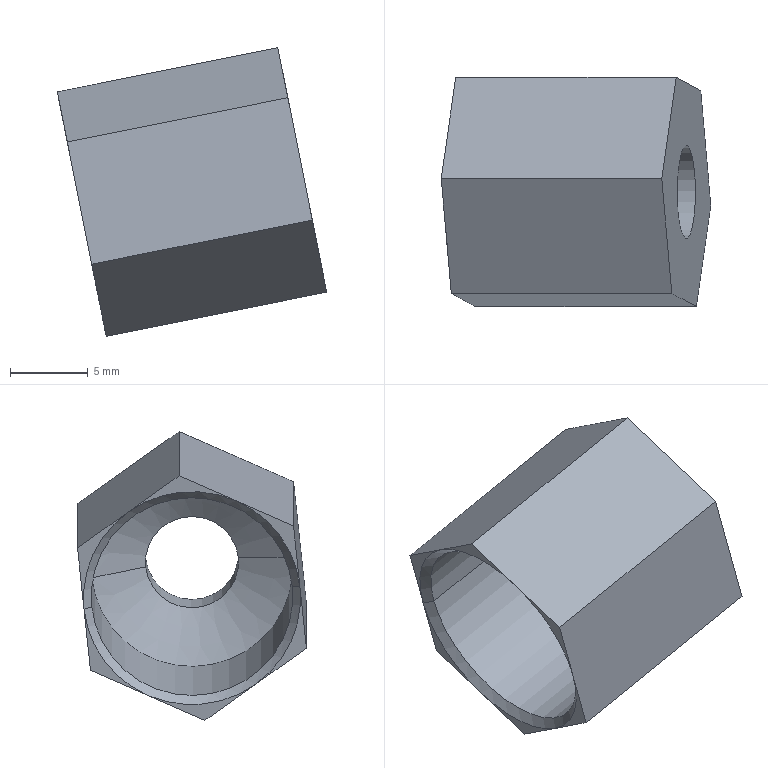Component | SolidWorks | 2-1 | 1 solid | 21 faces | box 17.38 x 14.76 x 18.62 mm | volume 920 mm3 | plane 13 | cone 4 | cylinder 4 | commonest cylinder face diameters 13 x2 6 x2
STEP:
#1=COLOUR_RGB('',0.7922,0.8196,0.9333);
#2=FILL_AREA_STYLE_COLOUR('',#1);
#3=FILL_AREA_STYLE('',(#2));
#4=SURFACE_STYLE_FILL_AREA(#3);
#5=SURFACE_SIDE_STYLE('',(#4));
#6=SURFACE_STYLE_USAGE(.BOTH.,#5);
#7=PRESENTATION_STYLE_ASSIGNMENT((#6));
#8=CARTESIAN_POINT('',(2.804,-12.312,0.535));
#9=VERTEX_POINT('',#8);
#10=CARTESIAN_POINT('',(2.793,-12.821,0.5869));
#11=VERTEX_POINT('',#10);
#12=CARTESIAN_POINT('',(2.799,-12.567,0.5609));
#13=DIRECTION('',(-0.9805,-0.,-0.1965));
#14=DIRECTION('',(-0.0203,-0.9947,0.1013));
#15=AXIS2_PLACEMENT_3D('',#12,#13,#14);
#16=CIRCLE('',#15,0.2559);
#17=EDGE_CURVE('',#9,#11,#16,.T.);
#18=ORIENTED_EDGE('',*,*,#17,.F.);
#19=CARTESIAN_POINT('',(2.785,-12.293,0.5292));
#20=VERTEX_POINT('',#19);
#21=CARTESIAN_POINT('',(2.804,-12.312,0.535));
#22=DIRECTION('',(-0.679,0.7033,-0.2106));
#23=VECTOR('',#22,39.37);
#24=LINE('',#21,#23);
#25=EDGE_CURVE('',#9,#20,#24,.T.);
#26=ORIENTED_EDGE('',*,*,#25,.T.);
#27=CARTESIAN_POINT('',(2.829,-12.455,0.3103));
#28=VERTEX_POINT('',#27);
#29=CARTESIAN_POINT('',(2.779,-12.567,0.5571));
#30=DIRECTION('',(0.9805,0.,0.1965));
#31=DIRECTION('',(-0.0203,-0.9947,0.1013));
#32=AXIS2_PLACEMENT_3D('',#29,#30,#31);
#33=CIRCLE('',#32,0.2756);
#34=EDGE_CURVE('',#28,#20,#33,.T.);
#35=ORIENTED_EDGE('',*,*,#34,.F.);
#36=CARTESIAN_POINT('',(2.823,-12.729,0.3383));
#37=VERTEX_POINT('',#36);
#38=CARTESIAN_POINT('',(2.779,-12.567,0.5571));
#39=DIRECTION('',(0.9805,0.,0.1965));
#40=DIRECTION('',(-0.0203,-0.9947,0.1013));
#41=AXIS2_PLACEMENT_3D('',#38,#39,#40);
#42=CIRCLE('',#41,0.2756);
#43=EDGE_CURVE('',#37,#28,#42,.T.);
#44=ORIENTED_EDGE('',*,*,#43,.F.);
#45=CARTESIAN_POINT('',(2.774,-12.841,0.585));
#46=VERTEX_POINT('',#45);
#47=CARTESIAN_POINT('',(2.779,-12.567,0.5571));
#48=DIRECTION('',(0.9805,0.,0.1965));
#49=DIRECTION('',(-0.0203,-0.9947,0.1013));
#50=AXIS2_PLACEMENT_3D('',#47,#48,#49);
#51=CIRCLE('',#50,0.2756);
#52=EDGE_CURVE('',#46,#37,#51,.T.);
#53=ORIENTED_EDGE('',*,*,#52,.F.);
#54=CARTESIAN_POINT('',(2.793,-12.821,0.5869));
#55=DIRECTION('',(-0.7077,-0.7033,-0.06734));
#56=VECTOR('',#55,39.37);
#57=LINE('',#54,#56);
#58=EDGE_CURVE('',#11,#46,#57,.T.);
#59=ORIENTED_EDGE('',*,*,#58,.F.);
#60=EDGE_LOOP('',(#18,#26,#35,#44,#53,#59));
#61=FACE_OUTER_BOUND('',#60,.T.);
#62=CARTESIAN_POINT('',(2.799,-12.567,0.5609));
#63=DIRECTION('',(-0.9805,-0.,-0.1965));
#64=DIRECTION('',(-0.0203,-0.9947,0.1013));
#65=AXIS2_PLACEMENT_3D('',#62,#63,#64);
#66=CONICAL_SURFACE('',#65,0.2559,0.7854);
#67=ADVANCED_FACE('',(#61),#66,.F.);
#68=CARTESIAN_POINT('',(3.171,-12.312,0.6085));
#69=VERTEX_POINT('',#68);
#70=CARTESIAN_POINT('',(3.16,-12.821,0.6604));
#71=VERTEX_POINT('',#70);
#72=CARTESIAN_POINT('',(3.165,-12.567,0.6344));
#73=DIRECTION('',(-0.9805,-0.,-0.1965));
#74=DIRECTION('',(-0.0203,-0.9947,0.1013));
#75=AXIS2_PLACEMENT_3D('',#72,#73,#74);
#76=CIRCLE('',#75,0.2559);
#77=EDGE_CURVE('',#69,#71,#76,.T.);
#78=ORIENTED_EDGE('',*,*,#77,.F.);
#79=CARTESIAN_POINT('',(2.785,-12.312,0.5311));
#80=DIRECTION('',(-0.9805,-0.,-0.1965));
#81=VECTOR('',#80,39.37);
#82=LINE('',#79,#81);
#83=EDGE_CURVE('',#69,#9,#82,.T.);
#84=ORIENTED_EDGE('',*,*,#83,.T.);
#85=ORIENTED_EDGE('',*,*,#17,.T.);
#86=CARTESIAN_POINT('',(2.774,-12.821,0.583));
#87=DIRECTION('',(-0.9805,-0.,-0.1965));
#88=VECTOR('',#87,39.37);
#89=LINE('',#86,#88);
#90=EDGE_CURVE('',#71,#11,#89,.T.);
#91=ORIENTED_EDGE('',*,*,#90,.F.);
#92=EDGE_LOOP('',(#78,#84,#85,#91));
#93=FACE_OUTER_BOUND('',#92,.T.);
#94=CARTESIAN_POINT('',(2.779,-12.567,0.5571));
#95=DIRECTION('',(-0.9805,-0.,-0.1965));
#96=DIRECTION('',(-0.0203,-0.9947,0.1013));
#97=AXIS2_PLACEMENT_3D('',#94,#95,#96);
#98=CYLINDRICAL_SURFACE('',#97,0.2559);
#99=ADVANCED_FACE('',(#93),#98,.F.);
#100=CARTESIAN_POINT('',(3.237,-12.449,0.6363));
#101=VERTEX_POINT('',#100);
#102=CARTESIAN_POINT('',(3.232,-12.684,0.6602));
#103=VERTEX_POINT('',#102);
#104=CARTESIAN_POINT('',(3.234,-12.567,0.6482));
#105=DIRECTION('',(-0.9805,-0.,-0.1965));
#106=DIRECTION('',(-0.0203,-0.9947,0.1013));
#107=AXIS2_PLACEMENT_3D('',#104,#105,#106);
#108=CIRCLE('',#107,0.1181);
#109=EDGE_CURVE('',#101,#103,#108,.T.);
#110=ORIENTED_EDGE('',*,*,#109,.F.);
#111=CARTESIAN_POINT('',(3.171,-12.312,0.6085));
#112=DIRECTION('',(-0.427,0.8862,-0.1795));
#113=VECTOR('',#112,39.37);
#114=LINE('',#111,#113);
#115=EDGE_CURVE('',#101,#69,#114,.T.);
#116=ORIENTED_EDGE('',*,*,#115,.T.);
#117=ORIENTED_EDGE('',*,*,#77,.T.);
#118=CARTESIAN_POINT('',(3.16,-12.821,0.6604));
#119=DIRECTION('',(-0.4632,-0.8862,0.001028));
#120=VECTOR('',#119,39.37);
#121=LINE('',#118,#120);
#122=EDGE_CURVE('',#103,#71,#121,.T.);
#123=ORIENTED_EDGE('',*,*,#122,.F.);
#124=EDGE_LOOP('',(#110,#116,#117,#123));
#125=FACE_OUTER_BOUND('',#124,.T.);
#126=CARTESIAN_POINT('',(3.165,-12.567,0.6344));
#127=DIRECTION('',(-0.9805,-0.,-0.1965));
#128=DIRECTION('',(-0.0203,-0.9947,0.1013));
#129=AXIS2_PLACEMENT_3D('',#126,#127,#128);
#130=CONICAL_SURFACE('',#129,0.2559,1.1);
#131=ADVANCED_FACE('',(#125),#130,.F.);
#132=CARTESIAN_POINT('',(3.342,-12.449,0.6573));
#133=VERTEX_POINT('',#132);
#134=CARTESIAN_POINT('',(3.337,-12.684,0.6812));
#135=VERTEX_POINT('',#134);
#136=CARTESIAN_POINT('',(3.339,-12.567,0.6693));
#137=DIRECTION('',(-0.9805,-0.,-0.1965));
#138=DIRECTION('',(-0.0203,-0.9947,0.1013));
#139=AXIS2_PLACEMENT_3D('',#136,#137,#138);
#140=CIRCLE('',#139,0.1181);
#141=EDGE_CURVE('',#133,#135,#140,.T.);
#142=ORIENTED_EDGE('',*,*,#141,.F.);
#143=CARTESIAN_POINT('',(2.782,-12.449,0.5451));
#144=DIRECTION('',(-0.9805,-0.,-0.1965));
#145=VECTOR('',#144,39.37);
#146=LINE('',#143,#145);
#147=EDGE_CURVE('',#133,#101,#146,.T.);
#148=ORIENTED_EDGE('',*,*,#147,.T.);
#149=ORIENTED_EDGE('',*,*,#109,.T.);
#150=CARTESIAN_POINT('',(2.777,-12.684,0.569));
#151=DIRECTION('',(-0.9805,-0.,-0.1965));
#152=VECTOR('',#151,39.37);
#153=LINE('',#150,#152);
#154=EDGE_CURVE('',#135,#103,#153,.T.);
#155=ORIENTED_EDGE('',*,*,#154,.F.);
#156=EDGE_LOOP('',(#142,#148,#149,#155));
#157=FACE_OUTER_BOUND('',#156,.T.);
#158=CARTESIAN_POINT('',(2.779,-12.567,0.5571));
#159=DIRECTION('',(-0.9805,-0.,-0.1965));
#160=DIRECTION('',(-0.0203,-0.9947,0.1013));
#161=AXIS2_PLACEMENT_3D('',#158,#159,#160);
#162=CYLINDRICAL_SURFACE('',#161,0.1181);
#163=ADVANCED_FACE('',(#157),#162,.F.);
#164=CARTESIAN_POINT('',(2.805,-12.857,0.4298));
#165=VERTEX_POINT('',#164);
#166=CARTESIAN_POINT('',(2.805,-12.857,0.4298));
#167=DIRECTION('',(-0.1955,0.1033,0.9753));
#168=VECTOR('',#167,39.37);
#169=LINE('',#166,#168);
#170=EDGE_CURVE('',#165,#46,#169,.T.);
#171=ORIENTED_EDGE('',*,*,#170,.T.);
#172=ORIENTED_EDGE('',*,*,#52,.T.);
#173=CARTESIAN_POINT('',(2.842,-12.6,0.2467));
#174=DIRECTION('',(-0.1153,-0.8097,0.5753));
#175=VECTOR('',#174,39.37);
#176=LINE('',#173,#175);
#177=EDGE_CURVE('',#37,#165,#176,.T.);
#178=ORIENTED_EDGE('',*,*,#177,.T.);
#179=EDGE_LOOP('',(#171,#172,#178));
#180=FACE_OUTER_BOUND('',#179,.T.);
#181=CARTESIAN_POINT('',(2.779,-12.567,0.5571));
#182=DIRECTION('',(-0.9805,-0.,-0.1965));
#183=DIRECTION('',(-0.0203,-0.9947,0.1013));
#184=AXIS2_PLACEMENT_3D('',#181,#182,#183);
#185=PLANE('',#184);
#186=ADVANCED_FACE('',(#180),#185,.T.);
#187=CARTESIAN_POINT('',(2.842,-12.6,0.2467));
#188=VERTEX_POINT('',#187);
#189=CARTESIAN_POINT('',(2.842,-12.6,0.2467));
#190=DIRECTION('',(-0.1153,-0.8097,0.5753));
#191=VECTOR('',#190,39.37);
#192=LINE('',#189,#191);
#193=EDGE_CURVE('',#188,#37,#192,.T.);
#194=ORIENTED_EDGE('',*,*,#193,.T.);
#195=ORIENTED_EDGE('',*,*,#43,.T.);
#196=CARTESIAN_POINT('',(2.816,-12.309,0.374));
#197=DIRECTION('',(0.08015,-0.913,-0.3999));
#198=VECTOR('',#197,39.37);
#199=LINE('',#196,#198);
#200=EDGE_CURVE('',#28,#188,#199,.T.);
#201=ORIENTED_EDGE('',*,*,#200,.T.);
#202=EDGE_LOOP('',(#194,#195,#201));
#203=FACE_OUTER_BOUND('',#202,.T.);
#204=CARTESIAN_POINT('',(2.779,-12.567,0.5571));
#205=DIRECTION('',(-0.9805,-0.,-0.1965));
#206=DIRECTION('',(-0.0203,-0.9947,0.1013));
#207=AXIS2_PLACEMENT_3D('',#204,#205,#206);
#208=PLANE('',#207);
#209=ADVANCED_FACE('',(#203),#208,.T.);
#210=CARTESIAN_POINT('',(2.816,-12.309,0.374));
#211=VERTEX_POINT('',#210);
#212=CARTESIAN_POINT('',(2.816,-12.309,0.374));
#213=DIRECTION('',(0.08015,-0.913,-0.3999));
#214=VECTOR('',#213,39.37);
#215=LINE('',#212,#214);
#216=EDGE_CURVE('',#211,#28,#215,.T.);
#217=ORIENTED_EDGE('',*,*,#216,.T.);
#218=ORIENTED_EDGE('',*,*,#34,.T.);
#219=CARTESIAN_POINT('',(2.754,-12.276,0.6843));
#220=DIRECTION('',(0.1955,-0.1033,-0.9753));
#221=VECTOR('',#220,39.37);
#222=LINE('',#219,#221);
#223=EDGE_CURVE('',#20,#211,#222,.T.);
#224=ORIENTED_EDGE('',*,*,#223,.T.);
#225=EDGE_LOOP('',(#217,#218,#224));
#226=FACE_OUTER_BOUND('',#225,.T.);
#227=CARTESIAN_POINT('',(2.779,-12.567,0.5571));
#228=DIRECTION('',(-0.9805,-0.,-0.1965));
#229=DIRECTION('',(-0.0203,-0.9947,0.1013));
#230=AXIS2_PLACEMENT_3D('',#227,#228,#229);
#231=PLANE('',#230);
#232=ADVANCED_FACE('',(#226),#231,.T.);
#233=CARTESIAN_POINT('',(2.754,-12.276,0.6843));
#234=VERTEX_POINT('',#233);
#235=CARTESIAN_POINT('',(2.754,-12.276,0.6843));
#236=DIRECTION('',(0.1955,-0.1033,-0.9753));
#237=VECTOR('',#236,39.37);
#238=LINE('',#235,#237);
#239=EDGE_CURVE('',#234,#20,#238,.T.);
#240=ORIENTED_EDGE('',*,*,#239,.T.);
#241=CARTESIAN_POINT('',(2.736,-12.405,0.7759));
#242=VERTEX_POINT('',#241);
#243=CARTESIAN_POINT('',(2.779,-12.567,0.5571));
#244=DIRECTION('',(0.9805,0.,0.1965));
#245=DIRECTION('',(-0.0203,-0.9947,0.1013));
#246=AXIS2_PLACEMENT_3D('',#243,#244,#245);
#247=CIRCLE('',#246,0.2756);
#248=EDGE_CURVE('',#20,#242,#247,.T.);
#249=ORIENTED_EDGE('',*,*,#248,.T.);
#250=CARTESIAN_POINT('',(2.717,-12.534,0.8674));
#251=DIRECTION('',(0.1153,0.8097,-0.5753));
#252=VECTOR('',#251,39.37);
#253=LINE('',#250,#252);
#254=EDGE_CURVE('',#242,#234,#253,.T.);
#255=ORIENTED_EDGE('',*,*,#254,.T.);
#256=EDGE_LOOP('',(#240,#249,#255));
#257=FACE_OUTER_BOUND('',#256,.T.);
#258=CARTESIAN_POINT('',(2.779,-12.567,0.5571));
#259=DIRECTION('',(-0.9805,-0.,-0.1965));
#260=DIRECTION('',(-0.0203,-0.9947,0.1013));
#261=AXIS2_PLACEMENT_3D('',#258,#259,#260);
#262=PLANE('',#261);
#263=ADVANCED_FACE('',(#257),#262,.T.);
#264=CARTESIAN_POINT('',(2.717,-12.534,0.8674));
#265=VERTEX_POINT('',#264);
#266=CARTESIAN_POINT('',(2.717,-12.534,0.8674));
#267=DIRECTION('',(0.1153,0.8097,-0.5753));
#268=VECTOR('',#267,39.37);
#269=LINE('',#266,#268);
#270=EDGE_CURVE('',#265,#242,#269,.T.);
#271=ORIENTED_EDGE('',*,*,#270,.T.);
#272=CARTESIAN_POINT('',(2.73,-12.679,0.8038));
#273=VERTEX_POINT('',#272);
#274=CARTESIAN_POINT('',(2.779,-12.567,0.5571));
#275=DIRECTION('',(0.9805,0.,0.1965));
#276=DIRECTION('',(-0.0203,-0.9947,0.1013));
#277=AXIS2_PLACEMENT_3D('',#274,#275,#276);
#278=CIRCLE('',#277,0.2756);
#279=EDGE_CURVE('',#242,#273,#278,.T.);
#280=ORIENTED_EDGE('',*,*,#279,.T.);
#281=CARTESIAN_POINT('',(2.743,-12.825,0.7402));
#282=DIRECTION('',(-0.08015,0.913,0.3999));
#283=VECTOR('',#282,39.37);
#284=LINE('',#281,#283);
#285=EDGE_CURVE('',#273,#265,#284,.T.);
#286=ORIENTED_EDGE('',*,*,#285,.T.);
#287=EDGE_LOOP('',(#271,#280,#286));
#288=FACE_OUTER_BOUND('',#287,.T.);
#289=CARTESIAN_POINT('',(2.779,-12.567,0.5571));
#290=DIRECTION('',(-0.9805,-0.,-0.1965));
#291=DIRECTION('',(-0.0203,-0.9947,0.1013));
#292=AXIS2_PLACEMENT_3D('',#289,#290,#291);
#293=PLANE('',#292);
#294=ADVANCED_FACE('',(#288),#293,.T.);
#295=CARTESIAN_POINT('',(3.277,-12.534,0.9796));
#296=VERTEX_POINT('',#295);
#297=CARTESIAN_POINT('',(3.314,-12.276,0.7965));
#298=VERTEX_POINT('',#297);
#299=CARTESIAN_POINT('',(3.277,-12.534,0.9796));
#300=DIRECTION('',(0.1153,0.8097,-0.5753));
#301=VECTOR('',#300,39.37);
#302=LINE('',#299,#301);
#303=EDGE_CURVE('',#296,#298,#302,.T.);
#304=ORIENTED_EDGE('',*,*,#303,.T.);
#305=CARTESIAN_POINT('',(2.754,-12.276,0.6843));
#306=DIRECTION('',(0.9805,0.,0.1965));
#307=VECTOR('',#306,39.37);
#308=LINE('',#305,#307);
#309=EDGE_CURVE('',#234,#298,#308,.T.);
#310=ORIENTED_EDGE('',*,*,#309,.F.);
#311=ORIENTED_EDGE('',*,*,#254,.F.);
#312=ORIENTED_EDGE('',*,*,#270,.F.);
#313=CARTESIAN_POINT('',(2.717,-12.534,0.8674));
#314=DIRECTION('',(0.9805,0.,0.1965));
#315=VECTOR('',#314,39.37);
#316=LINE('',#313,#315);
#317=EDGE_CURVE('',#265,#296,#316,.T.);
#318=ORIENTED_EDGE('',*,*,#317,.T.);
#319=EDGE_LOOP('',(#304,#310,#311,#312,#318));
#320=FACE_OUTER_BOUND('',#319,.T.);
#321=CARTESIAN_POINT('',(2.717,-12.534,0.8674));
#322=DIRECTION('',(0.1591,-0.5868,-0.794));
#323=DIRECTION('',(-0.1153,-0.8097,0.5753));
#324=AXIS2_PLACEMENT_3D('',#321,#322,#323);
#325=PLANE('',#324);
#326=ADVANCED_FACE('',(#320),#325,.F.);
#327=CARTESIAN_POINT('',(3.376,-12.309,0.4862));
#328=VERTEX_POINT('',#327);
#329=CARTESIAN_POINT('',(3.314,-12.276,0.7965));
#330=DIRECTION('',(0.1955,-0.1033,-0.9753));
#331=VECTOR('',#330,39.37);
#332=LINE('',#329,#331);
#333=EDGE_CURVE('',#298,#328,#332,.T.);
#334=ORIENTED_EDGE('',*,*,#333,.T.);
#335=CARTESIAN_POINT('',(2.816,-12.309,0.374));
#336=DIRECTION('',(0.9805,0.,0.1965));
#337=VECTOR('',#336,39.37);
#338=LINE('',#335,#337);
#339=EDGE_CURVE('',#211,#328,#338,.T.);
#340=ORIENTED_EDGE('',*,*,#339,.F.);
#341=ORIENTED_EDGE('',*,*,#223,.F.);
#342=ORIENTED_EDGE('',*,*,#239,.F.);
#343=ORIENTED_EDGE('',*,*,#309,.T.);
#344=EDGE_LOOP('',(#334,#340,#341,#342,#343));
#345=FACE_OUTER_BOUND('',#344,.T.);
#346=CARTESIAN_POINT('',(2.754,-12.276,0.6843));
#347=DIRECTION('',(-0.0203,-0.9947,0.1013));
#348=DIRECTION('',(-0.1955,0.1033,0.9753));
#349=AXIS2_PLACEMENT_3D('',#346,#347,#348);
#350=PLANE('',#349);
#351=ADVANCED_FACE('',(#345),#350,.F.);
#352=CARTESIAN_POINT('',(3.401,-12.6,0.3589));
#353=VERTEX_POINT('',#352);
#354=CARTESIAN_POINT('',(3.376,-12.309,0.4862));
#355=DIRECTION('',(0.08015,-0.913,-0.3999));
#356=VECTOR('',#355,39.37);
#357=LINE('',#354,#356);
#358=EDGE_CURVE('',#328,#353,#357,.T.);
#359=ORIENTED_EDGE('',*,*,#358,.T.);
#360=CARTESIAN_POINT('',(2.842,-12.6,0.2467));
#361=DIRECTION('',(0.9805,0.,0.1965));
#362=VECTOR('',#361,39.37);
#363=LINE('',#360,#362);
#364=EDGE_CURVE('',#188,#353,#363,.T.);
#365=ORIENTED_EDGE('',*,*,#364,.F.);
#366=ORIENTED_EDGE('',*,*,#200,.F.);
#367=ORIENTED_EDGE('',*,*,#216,.F.);
#368=ORIENTED_EDGE('',*,*,#339,.T.);
#369=EDGE_LOOP('',(#359,#365,#366,#367,#368));
#370=FACE_OUTER_BOUND('',#369,.T.);
#371=CARTESIAN_POINT('',(2.816,-12.309,0.374));
#372=DIRECTION('',(-0.1794,-0.4079,0.8952));
#373=DIRECTION('',(-0.08015,0.913,0.3999));
#374=AXIS2_PLACEMENT_3D('',#371,#372,#373);
#375=PLANE('',#374);
#376=ADVANCED_FACE('',(#370),#375,.F.);
#377=CARTESIAN_POINT('',(3.365,-12.857,0.542));
#378=VERTEX_POINT('',#377);
#379=CARTESIAN_POINT('',(3.401,-12.6,0.3589));
#380=DIRECTION('',(-0.1153,-0.8097,0.5753));
#381=VECTOR('',#380,39.37);
#382=LINE('',#379,#381);
#383=EDGE_CURVE('',#353,#378,#382,.T.);
#384=ORIENTED_EDGE('',*,*,#383,.T.);
#385=CARTESIAN_POINT('',(2.805,-12.857,0.4298));
#386=DIRECTION('',(0.9805,0.,0.1965));
#387=VECTOR('',#386,39.37);
#388=LINE('',#385,#387);
#389=EDGE_CURVE('',#165,#378,#388,.T.);
#390=ORIENTED_EDGE('',*,*,#389,.F.);
#391=ORIENTED_EDGE('',*,*,#177,.F.);
#392=ORIENTED_EDGE('',*,*,#193,.F.);
#393=ORIENTED_EDGE('',*,*,#364,.T.);
#394=EDGE_LOOP('',(#384,#390,#391,#392,#393));
#395=FACE_OUTER_BOUND('',#394,.T.);
#396=CARTESIAN_POINT('',(2.842,-12.6,0.2467));
#397=DIRECTION('',(-0.1591,0.5868,0.794));
#398=DIRECTION('',(0.1153,0.8097,-0.5753));
#399=AXIS2_PLACEMENT_3D('',#396,#397,#398);
#400=PLANE('',#399);
#401=ADVANCED_FACE('',(#395),#400,.F.);
#402=CARTESIAN_POINT('',(3.302,-12.825,0.8523));
#403=VERTEX_POINT('',#402);
#404=CARTESIAN_POINT('',(3.365,-12.857,0.542));
#405=DIRECTION('',(-0.1955,0.1033,0.9753));
#406=VECTOR('',#405,39.37);
#407=LINE('',#404,#406);
#408=EDGE_CURVE('',#378,#403,#407,.T.);
#409=ORIENTED_EDGE('',*,*,#408,.T.);
#410=CARTESIAN_POINT('',(2.743,-12.825,0.7402));
#411=VERTEX_POINT('',#410);
#412=CARTESIAN_POINT('',(2.743,-12.825,0.7402));
#413=DIRECTION('',(0.9805,0.,0.1965));
#414=VECTOR('',#413,39.37);
#415=LINE('',#412,#414);
#416=EDGE_CURVE('',#411,#403,#415,.T.);
#417=ORIENTED_EDGE('',*,*,#416,.F.);
#418=CARTESIAN_POINT('',(2.805,-12.857,0.4298));
#419=DIRECTION('',(-0.1955,0.1033,0.9753));
#420=VECTOR('',#419,39.37);
#421=LINE('',#418,#420);
#422=EDGE_CURVE('',#46,#411,#421,.T.);
#423=ORIENTED_EDGE('',*,*,#422,.F.);
#424=ORIENTED_EDGE('',*,*,#170,.F.);
#425=ORIENTED_EDGE('',*,*,#389,.T.);
#426=EDGE_LOOP('',(#409,#417,#423,#424,#425));
#427=FACE_OUTER_BOUND('',#426,.T.);
#428=CARTESIAN_POINT('',(2.805,-12.857,0.4298));
#429=DIRECTION('',(0.0203,0.9947,-0.1013));
#430=DIRECTION('',(0.1955,-0.1033,-0.9753));
#431=AXIS2_PLACEMENT_3D('',#428,#429,#430);
#432=PLANE('',#431);
#433=ADVANCED_FACE('',(#427),#432,.F.);
#434=CARTESIAN_POINT('',(3.302,-12.825,0.8523));
#435=DIRECTION('',(-0.08015,0.913,0.3999));
#436=VECTOR('',#435,39.37);
#437=LINE('',#434,#436);
#438=EDGE_CURVE('',#403,#296,#437,.T.);
#439=ORIENTED_EDGE('',*,*,#438,.T.);
#440=ORIENTED_EDGE('',*,*,#317,.F.);
#441=ORIENTED_EDGE('',*,*,#285,.F.);
#442=CARTESIAN_POINT('',(2.743,-12.825,0.7402));
#443=DIRECTION('',(-0.08015,0.913,0.3999));
#444=VECTOR('',#443,39.37);
#445=LINE('',#442,#444);
#446=EDGE_CURVE('',#411,#273,#445,.T.);
#447=ORIENTED_EDGE('',*,*,#446,.F.);
#448=ORIENTED_EDGE('',*,*,#416,.T.);
#449=EDGE_LOOP('',(#439,#440,#441,#447,#448));
#450=FACE_OUTER_BOUND('',#449,.T.);
#451=CARTESIAN_POINT('',(2.743,-12.825,0.7402));
#452=DIRECTION('',(0.1794,0.4079,-0.8952));
#453=DIRECTION('',(0.08015,-0.913,-0.3999));
#454=AXIS2_PLACEMENT_3D('',#451,#452,#453);
#455=PLANE('',#454);
#456=ADVANCED_FACE('',(#450),#455,.F.);
#457=ORIENTED_EDGE('',*,*,#446,.T.);
#458=CARTESIAN_POINT('',(2.779,-12.567,0.5571));
#459=DIRECTION('',(0.9805,0.,0.1965));
#460=DIRECTION('',(-0.0203,-0.9947,0.1013));
#461=AXIS2_PLACEMENT_3D('',#458,#459,#460);
#462=CIRCLE('',#461,0.2756);
#463=EDGE_CURVE('',#273,#46,#462,.T.);
#464=ORIENTED_EDGE('',*,*,#463,.T.);
#465=ORIENTED_EDGE('',*,*,#422,.T.);
#466=EDGE_LOOP('',(#457,#464,#465));
#467=FACE_OUTER_BOUND('',#466,.T.);
#468=CARTESIAN_POINT('',(2.779,-12.567,0.5571));
#469=DIRECTION('',(-0.9805,-0.,-0.1965));
#470=DIRECTION('',(-0.0203,-0.9947,0.1013));
#471=AXIS2_PLACEMENT_3D('',#468,#469,#470);
#472=PLANE('',#471);
#473=ADVANCED_FACE('',(#467),#472,.T.);
#474=CARTESIAN_POINT('',(3.339,-12.567,0.6693));
#475=DIRECTION('',(-0.9805,-0.,-0.1965));
#476=DIRECTION('',(-0.0203,-0.9947,0.1013));
#477=AXIS2_PLACEMENT_3D('',#474,#475,#476);
#478=CIRCLE('',#477,0.1181);
#479=EDGE_CURVE('',#135,#133,#478,.T.);
#480=ORIENTED_EDGE('',*,*,#479,.T.);
#481=ORIENTED_EDGE('',*,*,#141,.T.);
#482=EDGE_LOOP('',(#480,#481));
#483=FACE_BOUND('',#482,.T.);
#484=ORIENTED_EDGE('',*,*,#303,.F.);
#485=ORIENTED_EDGE('',*,*,#438,.F.);
#486=ORIENTED_EDGE('',*,*,#408,.F.);
#487=ORIENTED_EDGE('',*,*,#383,.F.);
#488=ORIENTED_EDGE('',*,*,#358,.F.);
#489=ORIENTED_EDGE('',*,*,#333,.F.);
#490=EDGE_LOOP('',(#484,#485,#486,#487,#488,#489));
#491=FACE_OUTER_BOUND('',#490,.T.);
#492=CARTESIAN_POINT('',(3.339,-12.567,0.6693));
#493=DIRECTION('',(-0.9805,-0.,-0.1965));
#494=DIRECTION('',(-0.0203,-0.9947,0.1013));
#495=AXIS2_PLACEMENT_3D('',#492,#493,#494);
#496=PLANE('',#495);
#497=ADVANCED_FACE('',(#483,#491),#496,.F.);
#498=ORIENTED_EDGE('',*,*,#147,.F.);
#499=ORIENTED_EDGE('',*,*,#479,.F.);
#500=ORIENTED_EDGE('',*,*,#154,.T.);
#501=CARTESIAN_POINT('',(3.234,-12.567,0.6482));
#502=DIRECTION('',(-0.9805,-0.,-0.1965));
#503=DIRECTION('',(-0.0203,-0.9947,0.1013));
#504=AXIS2_PLACEMENT_3D('',#501,#502,#503);
#505=CIRCLE('',#504,0.1181);
#506=EDGE_CURVE('',#103,#101,#505,.T.);
#507=ORIENTED_EDGE('',*,*,#506,.T.);
#508=EDGE_LOOP('',(#498,#499,#500,#507));
#509=FACE_OUTER_BOUND('',#508,.T.);
#510=CARTESIAN_POINT('',(2.779,-12.567,0.5571));
#511=DIRECTION('',(-0.9805,-0.,-0.1965));
#512=DIRECTION('',(-0.0203,-0.9947,0.1013));
#513=AXIS2_PLACEMENT_3D('',#510,#511,#512);
#514=CYLINDRICAL_SURFACE('',#513,0.1181);
#515=ADVANCED_FACE('',(#509),#514,.F.);
#516=ORIENTED_EDGE('',*,*,#115,.F.);
#517=ORIENTED_EDGE('',*,*,#506,.F.);
#518=ORIENTED_EDGE('',*,*,#122,.T.);
#519=CARTESIAN_POINT('',(3.165,-12.567,0.6344));
#520=DIRECTION('',(-0.9805,-0.,-0.1965));
#521=DIRECTION('',(-0.0203,-0.9947,0.1013));
#522=AXIS2_PLACEMENT_3D('',#519,#520,#521);
#523=CIRCLE('',#522,0.2559);
#524=EDGE_CURVE('',#71,#69,#523,.T.);
#525=ORIENTED_EDGE('',*,*,#524,.T.);
#526=EDGE_LOOP('',(#516,#517,#518,#525));
#527=FACE_OUTER_BOUND('',#526,.T.);
#528=CARTESIAN_POINT('',(3.165,-12.567,0.6344));
#529=DIRECTION('',(-0.9805,-0.,-0.1965));
#530=DIRECTION('',(-0.0203,-0.9947,0.1013));
#531=AXIS2_PLACEMENT_3D('',#528,#529,#530);
#532=CONICAL_SURFACE('',#531,0.2559,1.1);
#533=ADVANCED_FACE('',(#527),#532,.F.);
#534=ORIENTED_EDGE('',*,*,#83,.F.);
#535=ORIENTED_EDGE('',*,*,#524,.F.);
#536=ORIENTED_EDGE('',*,*,#90,.T.);
#537=CARTESIAN_POINT('',(2.799,-12.567,0.5609));
#538=DIRECTION('',(-0.9805,-0.,-0.1965));
#539=DIRECTION('',(-0.0203,-0.9947,0.1013));
#540=AXIS2_PLACEMENT_3D('',#537,#538,#539);
#541=CIRCLE('',#540,0.2559);
#542=EDGE_CURVE('',#11,#9,#541,.T.);
#543=ORIENTED_EDGE('',*,*,#542,.T.);
#544=EDGE_LOOP('',(#534,#535,#536,#543));
#545=FACE_OUTER_BOUND('',#544,.T.);
#546=CARTESIAN_POINT('',(2.779,-12.567,0.5571));
#547=DIRECTION('',(-0.9805,-0.,-0.1965));
#548=DIRECTION('',(-0.0203,-0.9947,0.1013));
#549=AXIS2_PLACEMENT_3D('',#546,#547,#548);
#550=CYLINDRICAL_SURFACE('',#549,0.2559);
#551=ADVANCED_FACE('',(#545),#550,.F.);
#552=ORIENTED_EDGE('',*,*,#25,.F.);
#553=ORIENTED_EDGE('',*,*,#542,.F.);
#554=ORIENTED_EDGE('',*,*,#58,.T.);
#555=ORIENTED_EDGE('',*,*,#463,.F.);
#556=ORIENTED_EDGE('',*,*,#279,.F.);
#557=ORIENTED_EDGE('',*,*,#248,.F.);
#558=EDGE_LOOP('',(#552,#553,#554,#555,#556,#557));
#559=FACE_OUTER_BOUND('',#558,.T.);
#560=CARTESIAN_POINT('',(2.799,-12.567,0.5609));
#561=DIRECTION('',(-0.9805,-0.,-0.1965));
#562=DIRECTION('',(-0.0203,-0.9947,0.1013));
#563=AXIS2_PLACEMENT_3D('',#560,#561,#562);
#564=CONICAL_SURFACE('',#563,0.2559,0.7854);
#565=ADVANCED_FACE('',(#559),#564,.F.);
#566=CLOSED_SHELL('',(#67,#99,#131,#163,#186,#209,#232,#263,#294,#326,#351,#376,#401,#433,#456,#473,#497,#515,#533,#551,#565));
#567=MANIFOLD_SOLID_BREP('',#566);
#568=STYLED_ITEM('',(#7),#567);
#569=PRESENTATION_LAYER_ASSIGNMENT('','',(#568));
#570=CARTESIAN_POINT('',(0.,0.,0.));
#571=DIRECTION('',(0.,0.,1.));
#572=DIRECTION('',(1.,0.,0.));
#573=AXIS2_PLACEMENT_3D('',#570,#571,#572);
#574=(LENGTH_UNIT()NAMED_UNIT(*)SI_UNIT($,.METRE.));
#575=LENGTH_MEASURE_WITH_UNIT(LENGTH_MEASURE(0.0254),#574);
#576=DIMENSIONAL_EXPONENTS(1.,0.,0.,0.,0.,0.,0.);
#577=(CONVERSION_BASED_UNIT('',#575)LENGTH_UNIT()NAMED_UNIT(#576));
#578=UNCERTAINTY_MEASURE_WITH_UNIT(LENGTH_MEASURE(0.00001),#577,'','');
#579=(NAMED_UNIT(*)PLANE_ANGLE_UNIT()SI_UNIT($,.RADIAN.));
#580=(NAMED_UNIT(*)SI_UNIT($,.STERADIAN.)SOLID_ANGLE_UNIT());
#581=(GEOMETRIC_REPRESENTATION_CONTEXT(3)GLOBAL_UNCERTAINTY_ASSIGNED_CONTEXT((#578))GLOBAL_UNIT_ASSIGNED_CONTEXT((#577,#579,#580))REPRESENTATION_CONTEXT('',''));
#582=ADVANCED_BREP_SHAPE_REPRESENTATION('',(#567,#573),#581);
#583=(LENGTH_UNIT()NAMED_UNIT(*)SI_UNIT($,.METRE.));
#584=LENGTH_MEASURE_WITH_UNIT(LENGTH_MEASURE(0.0254),#583);
#585=DIMENSIONAL_EXPONENTS(1.,0.,0.,0.,0.,0.,0.);
#586=(CONVERSION_BASED_UNIT('',#584)LENGTH_UNIT()NAMED_UNIT(#585));
#587=UNCERTAINTY_MEASURE_WITH_UNIT(LENGTH_MEASURE(0.00001),#586,'','');
#588=(NAMED_UNIT(*)PLANE_ANGLE_UNIT()SI_UNIT($,.RADIAN.));
#589=(NAMED_UNIT(*)SI_UNIT($,.STERADIAN.)SOLID_ANGLE_UNIT());
#590=(GEOMETRIC_REPRESENTATION_CONTEXT(3)GLOBAL_UNCERTAINTY_ASSIGNED_CONTEXT((#587))GLOBAL_UNIT_ASSIGNED_CONTEXT((#586,#588,#589))REPRESENTATION_CONTEXT('',''));
#591=MECHANICAL_DESIGN_GEOMETRIC_PRESENTATION_REPRESENTATION('',(#568),#590);